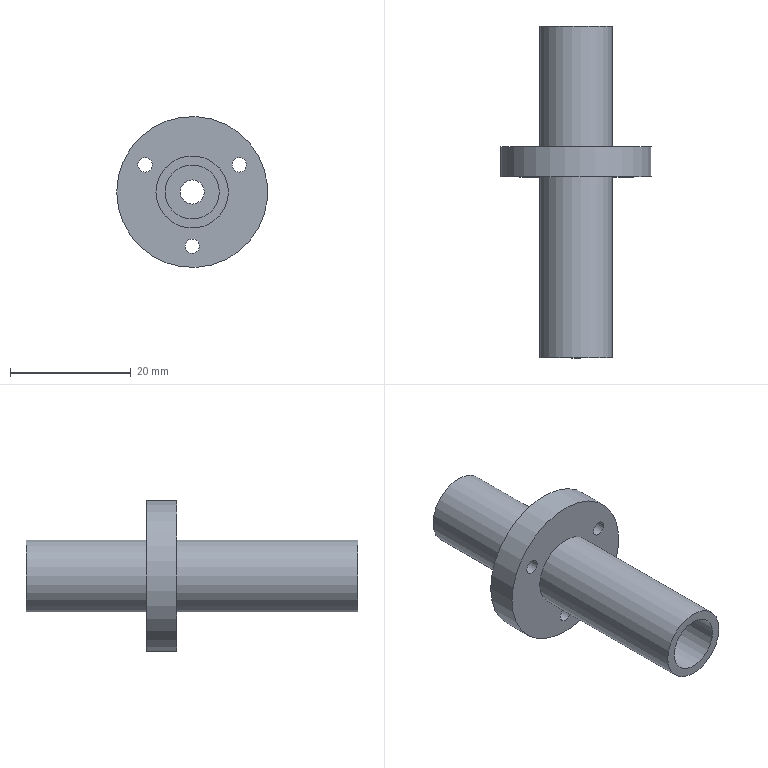Component | NX | SLEEVE | 1 solid | 19 faces | volume 5493 mm3 | cylinder 11 | plane 8 | commonest cylinder face diameters 2.4 x3 4.4 x3 12 x2 25 x1 9 x1 4 x1